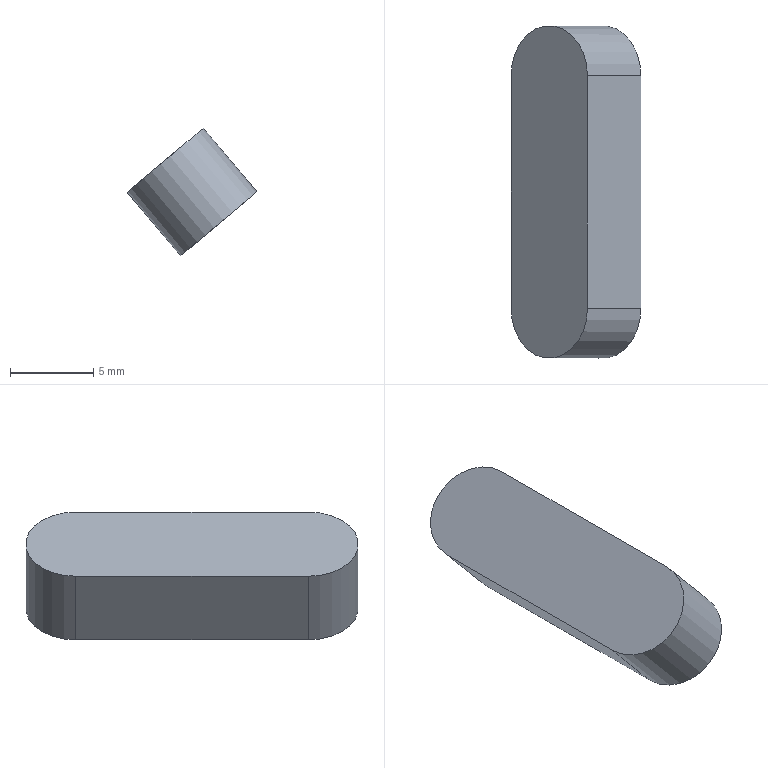Component | NX | KAMA | 1 solid | 6 faces | box 7.81 x 20 x 7.69 mm | volume 561 mm3 | plane 4 | cylinder 2 | commonest cylinder face diameters 6 x2
STEP:
#1=CARTESIAN_POINT('',(0.,0.,0.));
#2=DIRECTION('',(0.,0.,1.));
#3=DIRECTION('',(1.,0.,0.));
#4=AXIS2_PLACEMENT_3D('',#1,#2,#3);
#5=CARTESIAN_POINT('',(850.728,40.431,-87.047));
#6=VERTEX_POINT('',#5);
#7=CARTESIAN_POINT('',(850.728,26.431,-87.047));
#8=VERTEX_POINT('',#7);
#9=CARTESIAN_POINT('',(850.728,40.431,-87.047));
#10=DIRECTION('',(0.,-1.,0.));
#11=VECTOR('',#10,1.);
#12=LINE('',#9,#11);
#13=CARTESIAN_POINT('',(847.514,40.431,-83.217));
#14=DIRECTION('',(0.766,0.,0.6428));
#15=DIRECTION('',(0.6428,0.,-0.766));
#16=AXIS2_PLACEMENT_3D('',#13,#14,#15);
#17=PLANE('',#16);
#18=CARTESIAN_POINT('',(5.,0.));
#19=DIRECTION('',(0.,-1.));
#20=VECTOR('',#19,1.);
#21=LINE('',#18,#20);
#22=(GEOMETRIC_REPRESENTATION_CONTEXT(2)PARAMETRIC_REPRESENTATION_CONTEXT()REPRESENTATION_CONTEXT('',''));
#23=DEFINITIONAL_REPRESENTATION('',(#21),#22);
#24=PCURVE('',#17,#23);
#25=CARTESIAN_POINT('',(848.43,26.431,-88.975));
#26=DIRECTION('',(0.6428,0.,-0.766));
#27=DIRECTION('',(-0.766,0.,-0.6428));
#28=AXIS2_PLACEMENT_3D('',#25,#26,#27);
#29=PLANE('',#28);
#30=CARTESIAN_POINT('',(-3.,14.));
#31=DIRECTION('',(0.,-1.));
#32=VECTOR('',#31,1.);
#33=LINE('',#30,#32);
#34=(GEOMETRIC_REPRESENTATION_CONTEXT(2)PARAMETRIC_REPRESENTATION_CONTEXT()REPRESENTATION_CONTEXT('',''));
#35=DEFINITIONAL_REPRESENTATION('',(#33),#34);
#36=PCURVE('',#29,#35);
#37=SURFACE_CURVE('',#12,(#24,#36),.PCURVE_S1.);
#38=EDGE_CURVE('',#6,#8,#37,.T.);
#39=ORIENTED_EDGE('',*,*,#38,.F.);
#40=CARTESIAN_POINT('',(847.514,40.431,-83.217));
#41=VERTEX_POINT('',#40);
#42=CARTESIAN_POINT('',(847.514,40.431,-83.217));
#43=DIRECTION('',(0.6428,0.,-0.766));
#44=VECTOR('',#43,1.);
#45=LINE('',#42,#44);
#46=CARTESIAN_POINT('',(0.,0.));
#47=DIRECTION('',(1.,0.));
#48=VECTOR('',#47,1.);
#49=LINE('',#46,#48);
#50=(GEOMETRIC_REPRESENTATION_CONTEXT(2)PARAMETRIC_REPRESENTATION_CONTEXT()REPRESENTATION_CONTEXT('',''));
#51=DEFINITIONAL_REPRESENTATION('',(#49),#50);
#52=PCURVE('',#17,#51);
#53=CARTESIAN_POINT('',(845.216,40.431,-85.145));
#54=DIRECTION('',(0.6428,0.,-0.766));
#55=DIRECTION('',(-0.766,0.,-0.6428));
#56=AXIS2_PLACEMENT_3D('',#53,#54,#55);
#57=CYLINDRICAL_SURFACE('',#56,3.);
#58=CARTESIAN_POINT('',(3.142,0.));
#59=DIRECTION('',(0.,1.));
#60=VECTOR('',#59,1.);
#61=LINE('',#58,#60);
#62=(GEOMETRIC_REPRESENTATION_CONTEXT(2)PARAMETRIC_REPRESENTATION_CONTEXT()REPRESENTATION_CONTEXT('',''));
#63=DEFINITIONAL_REPRESENTATION('',(#61),#62);
#64=PCURVE('',#57,#63);
#65=SURFACE_CURVE('',#45,(#52,#64),.PCURVE_S1.);
#66=EDGE_CURVE('',#41,#6,#65,.T.);
#67=ORIENTED_EDGE('',*,*,#66,.F.);
#68=CARTESIAN_POINT('',(847.514,26.431,-83.217));
#69=VERTEX_POINT('',#68);
#70=CARTESIAN_POINT('',(847.514,40.431,-83.217));
#71=DIRECTION('',(0.,-1.,0.));
#72=VECTOR('',#71,1.);
#73=LINE('',#70,#72);
#74=CARTESIAN_POINT('',(0.,0.));
#75=DIRECTION('',(0.,-1.));
#76=VECTOR('',#75,1.);
#77=LINE('',#74,#76);
#78=(GEOMETRIC_REPRESENTATION_CONTEXT(2)PARAMETRIC_REPRESENTATION_CONTEXT()REPRESENTATION_CONTEXT('',''));
#79=DEFINITIONAL_REPRESENTATION('',(#77),#78);
#80=PCURVE('',#17,#79);
#81=CARTESIAN_POINT('',(845.216,26.431,-85.145));
#82=DIRECTION('',(0.6428,0.,-0.766));
#83=DIRECTION('',(-0.766,0.,-0.6428));
#84=AXIS2_PLACEMENT_3D('',#81,#82,#83);
#85=PLANE('',#84);
#86=CARTESIAN_POINT('',(-3.,14.));
#87=DIRECTION('',(0.,-1.));
#88=VECTOR('',#87,1.);
#89=LINE('',#86,#88);
#90=(GEOMETRIC_REPRESENTATION_CONTEXT(2)PARAMETRIC_REPRESENTATION_CONTEXT()REPRESENTATION_CONTEXT('',''));
#91=DEFINITIONAL_REPRESENTATION('',(#89),#90);
#92=PCURVE('',#85,#91);
#93=SURFACE_CURVE('',#73,(#80,#92),.PCURVE_S1.);
#94=EDGE_CURVE('',#41,#69,#93,.T.);
#95=ORIENTED_EDGE('',*,*,#94,.T.);
#96=CARTESIAN_POINT('',(847.514,26.431,-83.217));
#97=DIRECTION('',(0.6428,0.,-0.766));
#98=VECTOR('',#97,1.);
#99=LINE('',#96,#98);
#100=CARTESIAN_POINT('',(0.,-14.));
#101=DIRECTION('',(1.,0.));
#102=VECTOR('',#101,1.);
#103=LINE('',#100,#102);
#104=(GEOMETRIC_REPRESENTATION_CONTEXT(2)PARAMETRIC_REPRESENTATION_CONTEXT()REPRESENTATION_CONTEXT('',''));
#105=DEFINITIONAL_REPRESENTATION('',(#103),#104);
#106=PCURVE('',#17,#105);
#107=CARTESIAN_POINT('',(845.216,26.431,-85.145));
#108=DIRECTION('',(0.6428,0.,-0.766));
#109=DIRECTION('',(-0.766,0.,-0.6428));
#110=AXIS2_PLACEMENT_3D('',#107,#108,#109);
#111=CYLINDRICAL_SURFACE('',#110,3.);
#112=CARTESIAN_POINT('',(3.142,0.));
#113=DIRECTION('',(0.,1.));
#114=VECTOR('',#113,1.);
#115=LINE('',#112,#114);
#116=(GEOMETRIC_REPRESENTATION_CONTEXT(2)PARAMETRIC_REPRESENTATION_CONTEXT()REPRESENTATION_CONTEXT('',''));
#117=DEFINITIONAL_REPRESENTATION('',(#115),#116);
#118=PCURVE('',#111,#117);
#119=SURFACE_CURVE('',#99,(#106,#118),.PCURVE_S1.);
#120=EDGE_CURVE('',#69,#8,#119,.T.);
#121=ORIENTED_EDGE('',*,*,#120,.T.);
#122=EDGE_LOOP('',(#39,#67,#95,#121));
#123=FACE_BOUND('',#122,.T.);
#124=ADVANCED_FACE('',(#123),#17,.T.);
#125=CARTESIAN_POINT('',(846.132,26.431,-90.904));
#126=VERTEX_POINT('',#125);
#127=CARTESIAN_POINT('',(848.43,26.431,-88.975));
#128=DIRECTION('',(0.6428,0.,-0.766));
#129=DIRECTION('',(0.766,0.,0.6428));
#130=AXIS2_PLACEMENT_3D('',#127,#128,#129);
#131=CIRCLE('',#130,3.);
#132=CARTESIAN_POINT('',(3.142,5.));
#133=DIRECTION('',(1.,-0.));
#134=VECTOR('',#133,1.);
#135=LINE('',#132,#134);
#136=(GEOMETRIC_REPRESENTATION_CONTEXT(2)PARAMETRIC_REPRESENTATION_CONTEXT()REPRESENTATION_CONTEXT('',''));
#137=DEFINITIONAL_REPRESENTATION('',(#135),#136);
#138=PCURVE('',#111,#137);
#139=CARTESIAN_POINT('',(0.,0.));
#140=DIRECTION('',(-1.,0.));
#141=AXIS2_PLACEMENT_2D('',#139,#140);
#142=CIRCLE('',#141,3.);
#143=(GEOMETRIC_REPRESENTATION_CONTEXT(2)PARAMETRIC_REPRESENTATION_CONTEXT()REPRESENTATION_CONTEXT('',''));
#144=DEFINITIONAL_REPRESENTATION('',(#142),#143);
#145=PCURVE('',#29,#144);
#146=SURFACE_CURVE('',#131,(#138,#145),.PCURVE_S1.);
#147=EDGE_CURVE('',#8,#126,#146,.T.);
#148=ORIENTED_EDGE('',*,*,#147,.F.);
#149=ORIENTED_EDGE('',*,*,#120,.F.);
#150=CARTESIAN_POINT('',(842.918,26.431,-87.074));
#151=VERTEX_POINT('',#150);
#152=CARTESIAN_POINT('',(845.216,26.431,-85.145));
#153=DIRECTION('',(0.6428,0.,-0.766));
#154=DIRECTION('',(0.766,0.,0.6428));
#155=AXIS2_PLACEMENT_3D('',#152,#153,#154);
#156=CIRCLE('',#155,3.);
#157=CARTESIAN_POINT('',(3.142,0.));
#158=DIRECTION('',(1.,-0.));
#159=VECTOR('',#158,1.);
#160=LINE('',#157,#159);
#161=(GEOMETRIC_REPRESENTATION_CONTEXT(2)PARAMETRIC_REPRESENTATION_CONTEXT()REPRESENTATION_CONTEXT('',''));
#162=DEFINITIONAL_REPRESENTATION('',(#160),#161);
#163=PCURVE('',#111,#162);
#164=CARTESIAN_POINT('',(0.,0.));
#165=DIRECTION('',(-1.,0.));
#166=AXIS2_PLACEMENT_2D('',#164,#165);
#167=CIRCLE('',#166,3.);
#168=(GEOMETRIC_REPRESENTATION_CONTEXT(2)PARAMETRIC_REPRESENTATION_CONTEXT()REPRESENTATION_CONTEXT('',''));
#169=DEFINITIONAL_REPRESENTATION('',(#167),#168);
#170=PCURVE('',#85,#169);
#171=SURFACE_CURVE('',#156,(#163,#170),.PCURVE_S1.);
#172=EDGE_CURVE('',#69,#151,#171,.T.);
#173=ORIENTED_EDGE('',*,*,#172,.T.);
#174=CARTESIAN_POINT('',(842.918,26.431,-87.074));
#175=DIRECTION('',(0.6428,0.,-0.766));
#176=VECTOR('',#175,1.);
#177=LINE('',#174,#176);
#178=CARTESIAN_POINT('',(6.283,0.));
#179=DIRECTION('',(0.,1.));
#180=VECTOR('',#179,1.);
#181=LINE('',#178,#180);
#182=(GEOMETRIC_REPRESENTATION_CONTEXT(2)PARAMETRIC_REPRESENTATION_CONTEXT()REPRESENTATION_CONTEXT('',''));
#183=DEFINITIONAL_REPRESENTATION('',(#181),#182);
#184=PCURVE('',#111,#183);
#185=CARTESIAN_POINT('',(842.918,26.431,-87.074));
#186=DIRECTION('',(-0.766,0.,-0.6428));
#187=DIRECTION('',(-0.6428,0.,0.766));
#188=AXIS2_PLACEMENT_3D('',#185,#186,#187);
#189=PLANE('',#188);
#190=CARTESIAN_POINT('',(0.,0.));
#191=DIRECTION('',(-1.,0.));
#192=VECTOR('',#191,1.);
#193=LINE('',#190,#192);
#194=(GEOMETRIC_REPRESENTATION_CONTEXT(2)PARAMETRIC_REPRESENTATION_CONTEXT()REPRESENTATION_CONTEXT('',''));
#195=DEFINITIONAL_REPRESENTATION('',(#193),#194);
#196=PCURVE('',#189,#195);
#197=SURFACE_CURVE('',#177,(#184,#196),.PCURVE_S1.);
#198=EDGE_CURVE('',#151,#126,#197,.T.);
#199=ORIENTED_EDGE('',*,*,#198,.T.);
#200=EDGE_LOOP('',(#148,#149,#173,#199));
#201=FACE_BOUND('',#200,.T.);
#202=ADVANCED_FACE('',(#201),#111,.T.);
#203=CARTESIAN_POINT('',(846.132,40.431,-90.904));
#204=VERTEX_POINT('',#203);
#205=CARTESIAN_POINT('',(846.132,26.431,-90.904));
#206=DIRECTION('',(0.,1.,0.));
#207=VECTOR('',#206,1.);
#208=LINE('',#205,#207);
#209=CARTESIAN_POINT('',(-5.,0.));
#210=DIRECTION('',(0.,1.));
#211=VECTOR('',#210,1.);
#212=LINE('',#209,#211);
#213=(GEOMETRIC_REPRESENTATION_CONTEXT(2)PARAMETRIC_REPRESENTATION_CONTEXT()REPRESENTATION_CONTEXT('',''));
#214=DEFINITIONAL_REPRESENTATION('',(#212),#213);
#215=PCURVE('',#189,#214);
#216=CARTESIAN_POINT('',(3.,0.));
#217=DIRECTION('',(0.,1.));
#218=VECTOR('',#217,1.);
#219=LINE('',#216,#218);
#220=(GEOMETRIC_REPRESENTATION_CONTEXT(2)PARAMETRIC_REPRESENTATION_CONTEXT()REPRESENTATION_CONTEXT('',''));
#221=DEFINITIONAL_REPRESENTATION('',(#219),#220);
#222=PCURVE('',#29,#221);
#223=SURFACE_CURVE('',#208,(#215,#222),.PCURVE_S1.);
#224=EDGE_CURVE('',#126,#204,#223,.T.);
#225=ORIENTED_EDGE('',*,*,#224,.F.);
#226=ORIENTED_EDGE('',*,*,#198,.F.);
#227=CARTESIAN_POINT('',(842.918,40.431,-87.074));
#228=VERTEX_POINT('',#227);
#229=CARTESIAN_POINT('',(842.918,26.431,-87.074));
#230=DIRECTION('',(0.,1.,0.));
#231=VECTOR('',#230,1.);
#232=LINE('',#229,#231);
#233=CARTESIAN_POINT('',(0.,0.));
#234=DIRECTION('',(0.,1.));
#235=VECTOR('',#234,1.);
#236=LINE('',#233,#235);
#237=(GEOMETRIC_REPRESENTATION_CONTEXT(2)PARAMETRIC_REPRESENTATION_CONTEXT()REPRESENTATION_CONTEXT('',''));
#238=DEFINITIONAL_REPRESENTATION('',(#236),#237);
#239=PCURVE('',#189,#238);
#240=CARTESIAN_POINT('',(3.,0.));
#241=DIRECTION('',(0.,1.));
#242=VECTOR('',#241,1.);
#243=LINE('',#240,#242);
#244=(GEOMETRIC_REPRESENTATION_CONTEXT(2)PARAMETRIC_REPRESENTATION_CONTEXT()REPRESENTATION_CONTEXT('',''));
#245=DEFINITIONAL_REPRESENTATION('',(#243),#244);
#246=PCURVE('',#85,#245);
#247=SURFACE_CURVE('',#232,(#239,#246),.PCURVE_S1.);
#248=EDGE_CURVE('',#151,#228,#247,.T.);
#249=ORIENTED_EDGE('',*,*,#248,.T.);
#250=CARTESIAN_POINT('',(842.918,40.431,-87.074));
#251=DIRECTION('',(0.6428,0.,-0.766));
#252=VECTOR('',#251,1.);
#253=LINE('',#250,#252);
#254=CARTESIAN_POINT('',(0.,14.));
#255=DIRECTION('',(-1.,0.));
#256=VECTOR('',#255,1.);
#257=LINE('',#254,#256);
#258=(GEOMETRIC_REPRESENTATION_CONTEXT(2)PARAMETRIC_REPRESENTATION_CONTEXT()REPRESENTATION_CONTEXT('',''));
#259=DEFINITIONAL_REPRESENTATION('',(#257),#258);
#260=PCURVE('',#189,#259);
#261=CARTESIAN_POINT('',(0.,0.));
#262=DIRECTION('',(0.,1.));
#263=VECTOR('',#262,1.);
#264=LINE('',#261,#263);
#265=(GEOMETRIC_REPRESENTATION_CONTEXT(2)PARAMETRIC_REPRESENTATION_CONTEXT()REPRESENTATION_CONTEXT('',''));
#266=DEFINITIONAL_REPRESENTATION('',(#264),#265);
#267=PCURVE('',#57,#266);
#268=SURFACE_CURVE('',#253,(#260,#267),.PCURVE_S1.);
#269=EDGE_CURVE('',#228,#204,#268,.T.);
#270=ORIENTED_EDGE('',*,*,#269,.T.);
#271=EDGE_LOOP('',(#225,#226,#249,#270));
#272=FACE_BOUND('',#271,.T.);
#273=ADVANCED_FACE('',(#272),#189,.T.);
#274=CARTESIAN_POINT('',(848.43,40.431,-88.975));
#275=DIRECTION('',(0.6428,0.,-0.766));
#276=DIRECTION('',(0.766,0.,0.6428));
#277=AXIS2_PLACEMENT_3D('',#274,#275,#276);
#278=CIRCLE('',#277,3.);
#279=CARTESIAN_POINT('',(-3.142,5.));
#280=DIRECTION('',(1.,0.));
#281=VECTOR('',#280,1.);
#282=LINE('',#279,#281);
#283=(GEOMETRIC_REPRESENTATION_CONTEXT(2)PARAMETRIC_REPRESENTATION_CONTEXT()REPRESENTATION_CONTEXT('',''));
#284=DEFINITIONAL_REPRESENTATION('',(#282),#283);
#285=PCURVE('',#57,#284);
#286=CARTESIAN_POINT('',(0.,14.));
#287=DIRECTION('',(-1.,0.));
#288=AXIS2_PLACEMENT_2D('',#286,#287);
#289=CIRCLE('',#288,3.);
#290=(GEOMETRIC_REPRESENTATION_CONTEXT(2)PARAMETRIC_REPRESENTATION_CONTEXT()REPRESENTATION_CONTEXT('',''));
#291=DEFINITIONAL_REPRESENTATION('',(#289),#290);
#292=PCURVE('',#29,#291);
#293=SURFACE_CURVE('',#278,(#285,#292),.PCURVE_S1.);
#294=EDGE_CURVE('',#204,#6,#293,.T.);
#295=ORIENTED_EDGE('',*,*,#294,.F.);
#296=ORIENTED_EDGE('',*,*,#269,.F.);
#297=CARTESIAN_POINT('',(845.216,40.431,-85.145));
#298=DIRECTION('',(0.6428,0.,-0.766));
#299=DIRECTION('',(0.766,0.,0.6428));
#300=AXIS2_PLACEMENT_3D('',#297,#298,#299);
#301=CIRCLE('',#300,3.);
#302=CARTESIAN_POINT('',(-3.142,-0.));
#303=DIRECTION('',(1.,0.));
#304=VECTOR('',#303,1.);
#305=LINE('',#302,#304);
#306=(GEOMETRIC_REPRESENTATION_CONTEXT(2)PARAMETRIC_REPRESENTATION_CONTEXT()REPRESENTATION_CONTEXT('',''));
#307=DEFINITIONAL_REPRESENTATION('',(#305),#306);
#308=PCURVE('',#57,#307);
#309=CARTESIAN_POINT('',(0.,14.));
#310=DIRECTION('',(-1.,0.));
#311=AXIS2_PLACEMENT_2D('',#309,#310);
#312=CIRCLE('',#311,3.);
#313=(GEOMETRIC_REPRESENTATION_CONTEXT(2)PARAMETRIC_REPRESENTATION_CONTEXT()REPRESENTATION_CONTEXT('',''));
#314=DEFINITIONAL_REPRESENTATION('',(#312),#313);
#315=PCURVE('',#85,#314);
#316=SURFACE_CURVE('',#301,(#308,#315),.PCURVE_S1.);
#317=EDGE_CURVE('',#228,#41,#316,.T.);
#318=ORIENTED_EDGE('',*,*,#317,.T.);
#319=ORIENTED_EDGE('',*,*,#66,.T.);
#320=EDGE_LOOP('',(#295,#296,#318,#319));
#321=FACE_BOUND('',#320,.T.);
#322=ADVANCED_FACE('',(#321),#57,.T.);
#323=ORIENTED_EDGE('',*,*,#94,.F.);
#324=ORIENTED_EDGE('',*,*,#317,.F.);
#325=ORIENTED_EDGE('',*,*,#248,.F.);
#326=ORIENTED_EDGE('',*,*,#172,.F.);
#327=EDGE_LOOP('',(#323,#324,#325,#326));
#328=FACE_BOUND('',#327,.T.);
#329=ADVANCED_FACE('',(#328),#85,.F.);
#330=ORIENTED_EDGE('',*,*,#38,.T.);
#331=ORIENTED_EDGE('',*,*,#147,.T.);
#332=ORIENTED_EDGE('',*,*,#224,.T.);
#333=ORIENTED_EDGE('',*,*,#294,.T.);
#334=EDGE_LOOP('',(#330,#331,#332,#333));
#335=FACE_BOUND('',#334,.T.);
#336=ADVANCED_FACE('',(#335),#29,.T.);
#337=CLOSED_SHELL('',(#124,#202,#273,#322,#329,#336));
#338=MANIFOLD_SOLID_BREP('',#337);
#339=(LENGTH_UNIT()NAMED_UNIT(*)SI_UNIT(.MILLI.,.METRE.));
#340=UNCERTAINTY_MEASURE_WITH_UNIT(LENGTH_MEASURE(0.0000001),#339,'','');
#341=(NAMED_UNIT(*)PLANE_ANGLE_UNIT()SI_UNIT($,.RADIAN.));
#342=(NAMED_UNIT(*)SI_UNIT($,.STERADIAN.)SOLID_ANGLE_UNIT());
#343=(GEOMETRIC_REPRESENTATION_CONTEXT(3)GLOBAL_UNCERTAINTY_ASSIGNED_CONTEXT((#340))GLOBAL_UNIT_ASSIGNED_CONTEXT((#339,#341,#342))REPRESENTATION_CONTEXT('',''));
#344=ADVANCED_BREP_SHAPE_REPRESENTATION('',(#4,#338),#343);